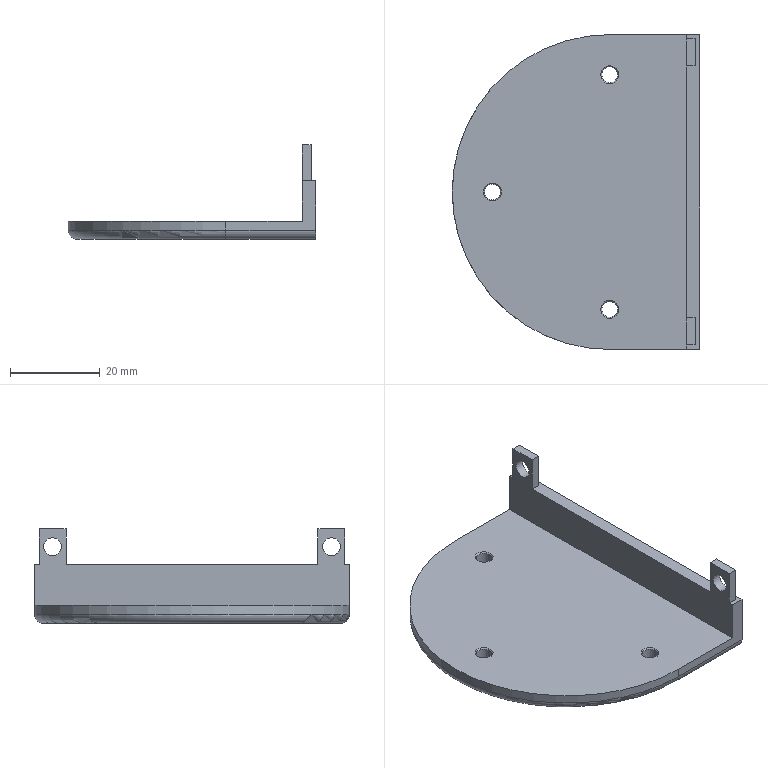Component | NX | FIXED | 1 solid | 30 faces | volume 15084 mm3 | plane 15 | cylinder 8 | cone 6 | torus 1 | commonest cylinder face diameters 4 x4 3.5 x3 70 x1